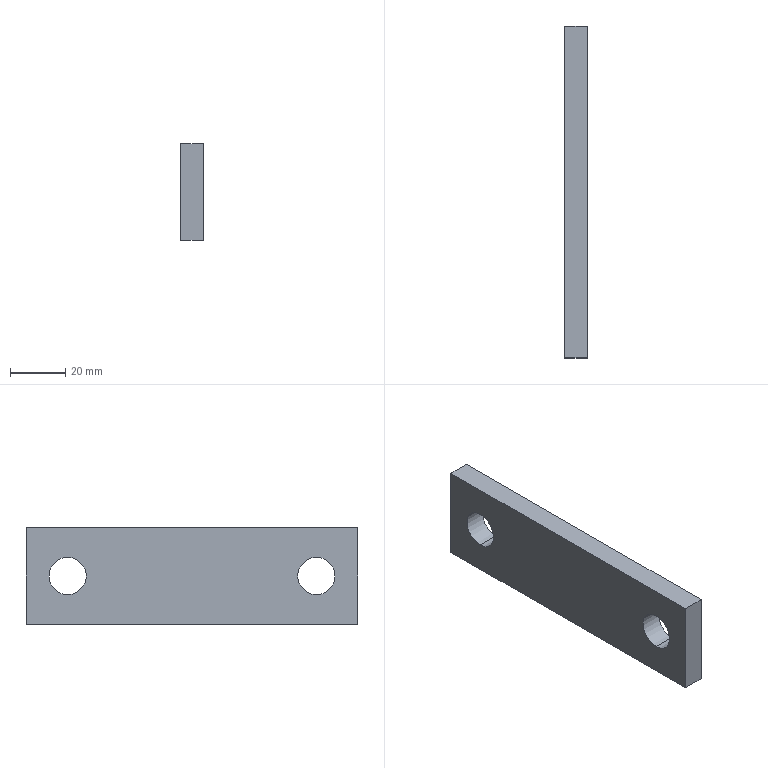Component | SolidWorks | BearingHousing-1_ShaftBaffle-1 | 1 solid | 10 faces | box 8 x 120 x 35 mm | volume 31310 mm3 | plane 6 | cylinder 4 | commonest cylinder face diameters 13.5 x4 | material Plain Carbon Steel
STEP:
#1=CARTESIAN_POINT('',(427.659,129.202,273.063));
#2=VERTEX_POINT('',#1);
#3=CARTESIAN_POINT('',(427.659,129.202,273.594));
#4=VERTEX_POINT('',#3);
#5=CARTESIAN_POINT('',(427.659,129.202,273.328));
#6=DIRECTION('',(-1.,-0.,0.));
#7=DIRECTION('',(0.,0.,1.));
#8=AXIS2_PLACEMENT_3D('',#5,#6,#7);
#9=CIRCLE('',#8,0.2657);
#10=EDGE_CURVE('',#2,#4,#9,.T.);
#11=ORIENTED_EDGE('',*,*,#10,.F.);
#12=CARTESIAN_POINT('',(427.344,129.202,273.063));
#13=VERTEX_POINT('',#12);
#14=CARTESIAN_POINT('',(427.659,129.202,273.063));
#15=DIRECTION('',(-1.,-0.,0.));
#16=VECTOR('',#15,39.37);
#17=LINE('',#14,#16);
#18=EDGE_CURVE('',#2,#13,#17,.T.);
#19=ORIENTED_EDGE('',*,*,#18,.T.);
#20=CARTESIAN_POINT('',(427.344,129.202,273.594));
#21=VERTEX_POINT('',#20);
#22=CARTESIAN_POINT('',(427.344,129.202,273.328));
#23=DIRECTION('',(-1.,-0.,0.));
#24=DIRECTION('',(0.,0.,1.));
#25=AXIS2_PLACEMENT_3D('',#22,#23,#24);
#26=CIRCLE('',#25,0.2657);
#27=EDGE_CURVE('',#13,#21,#26,.T.);
#28=ORIENTED_EDGE('',*,*,#27,.T.);
#29=CARTESIAN_POINT('',(427.659,129.202,273.594));
#30=DIRECTION('',(-1.,-0.,0.));
#31=VECTOR('',#30,39.37);
#32=LINE('',#29,#31);
#33=EDGE_CURVE('',#4,#21,#32,.T.);
#34=ORIENTED_EDGE('',*,*,#33,.F.);
#35=EDGE_LOOP('',(#11,#19,#28,#34));
#36=FACE_OUTER_BOUND('',#35,.T.);
#37=CARTESIAN_POINT('',(427.659,129.202,273.328));
#38=DIRECTION('',(-1.,-0.,0.));
#39=DIRECTION('',(0.,0.,1.));
#40=AXIS2_PLACEMENT_3D('',#37,#38,#39);
#41=CYLINDRICAL_SURFACE('',#40,0.2657);
#42=ADVANCED_FACE('',(#36),#41,.F.);
#43=CARTESIAN_POINT('',(427.659,125.659,273.063));
#44=VERTEX_POINT('',#43);
#45=CARTESIAN_POINT('',(427.659,125.659,273.594));
#46=VERTEX_POINT('',#45);
#47=CARTESIAN_POINT('',(427.659,125.659,273.328));
#48=DIRECTION('',(-1.,-0.,0.));
#49=DIRECTION('',(0.,0.,1.));
#50=AXIS2_PLACEMENT_3D('',#47,#48,#49);
#51=CIRCLE('',#50,0.2657);
#52=EDGE_CURVE('',#44,#46,#51,.T.);
#53=ORIENTED_EDGE('',*,*,#52,.F.);
#54=CARTESIAN_POINT('',(427.344,125.659,273.063));
#55=VERTEX_POINT('',#54);
#56=CARTESIAN_POINT('',(427.659,125.659,273.063));
#57=DIRECTION('',(-1.,-0.,0.));
#58=VECTOR('',#57,39.37);
#59=LINE('',#56,#58);
#60=EDGE_CURVE('',#44,#55,#59,.T.);
#61=ORIENTED_EDGE('',*,*,#60,.T.);
#62=CARTESIAN_POINT('',(427.344,125.659,273.594));
#63=VERTEX_POINT('',#62);
#64=CARTESIAN_POINT('',(427.344,125.659,273.328));
#65=DIRECTION('',(-1.,-0.,0.));
#66=DIRECTION('',(0.,0.,1.));
#67=AXIS2_PLACEMENT_3D('',#64,#65,#66);
#68=CIRCLE('',#67,0.2657);
#69=EDGE_CURVE('',#55,#63,#68,.T.);
#70=ORIENTED_EDGE('',*,*,#69,.T.);
#71=CARTESIAN_POINT('',(427.659,125.659,273.594));
#72=DIRECTION('',(-1.,-0.,0.));
#73=VECTOR('',#72,39.37);
#74=LINE('',#71,#73);
#75=EDGE_CURVE('',#46,#63,#74,.T.);
#76=ORIENTED_EDGE('',*,*,#75,.F.);
#77=EDGE_LOOP('',(#53,#61,#70,#76));
#78=FACE_OUTER_BOUND('',#77,.T.);
#79=CARTESIAN_POINT('',(427.659,125.659,273.328));
#80=DIRECTION('',(-1.,-0.,0.));
#81=DIRECTION('',(0.,0.,1.));
#82=AXIS2_PLACEMENT_3D('',#79,#80,#81);
#83=CYLINDRICAL_SURFACE('',#82,0.2657);
#84=ADVANCED_FACE('',(#78),#83,.F.);
#85=CARTESIAN_POINT('',(427.344,125.068,272.639));
#86=VERTEX_POINT('',#85);
#87=CARTESIAN_POINT('',(427.344,125.068,274.017));
#88=VERTEX_POINT('',#87);
#89=CARTESIAN_POINT('',(427.344,125.068,272.639));
#90=DIRECTION('',(-0.,0.,1.));
#91=VECTOR('',#90,39.37);
#92=LINE('',#89,#91);
#93=EDGE_CURVE('',#86,#88,#92,.T.);
#94=ORIENTED_EDGE('',*,*,#93,.F.);
#95=CARTESIAN_POINT('',(427.659,125.068,272.639));
#96=VERTEX_POINT('',#95);
#97=CARTESIAN_POINT('',(427.659,125.068,272.639));
#98=DIRECTION('',(-1.,-0.,0.));
#99=VECTOR('',#98,39.37);
#100=LINE('',#97,#99);
#101=EDGE_CURVE('',#96,#86,#100,.T.);
#102=ORIENTED_EDGE('',*,*,#101,.F.);
#103=CARTESIAN_POINT('',(427.659,125.068,274.017));
#104=VERTEX_POINT('',#103);
#105=CARTESIAN_POINT('',(427.659,125.068,272.639));
#106=DIRECTION('',(-0.,0.,1.));
#107=VECTOR('',#106,39.37);
#108=LINE('',#105,#107);
#109=EDGE_CURVE('',#96,#104,#108,.T.);
#110=ORIENTED_EDGE('',*,*,#109,.T.);
#111=CARTESIAN_POINT('',(427.659,125.068,274.017));
#112=DIRECTION('',(-1.,-0.,0.));
#113=VECTOR('',#112,39.37);
#114=LINE('',#111,#113);
#115=EDGE_CURVE('',#104,#88,#114,.T.);
#116=ORIENTED_EDGE('',*,*,#115,.T.);
#117=EDGE_LOOP('',(#94,#102,#110,#116));
#118=FACE_OUTER_BOUND('',#117,.T.);
#119=CARTESIAN_POINT('',(427.659,125.068,272.639));
#120=DIRECTION('',(0.,-1.,0.));
#121=DIRECTION('',(-0.,0.,1.));
#122=AXIS2_PLACEMENT_3D('',#119,#120,#121);
#123=PLANE('',#122);
#124=ADVANCED_FACE('',(#118),#123,.T.);
#125=CARTESIAN_POINT('',(427.344,129.793,272.639));
#126=VERTEX_POINT('',#125);
#127=CARTESIAN_POINT('',(427.344,125.068,272.639));
#128=DIRECTION('',(0.,-1.,0.));
#129=VECTOR('',#128,39.37);
#130=LINE('',#127,#129);
#131=EDGE_CURVE('',#126,#86,#130,.T.);
#132=ORIENTED_EDGE('',*,*,#131,.F.);
#133=CARTESIAN_POINT('',(427.659,129.793,272.639));
#134=VERTEX_POINT('',#133);
#135=CARTESIAN_POINT('',(427.659,129.793,272.639));
#136=DIRECTION('',(-1.,-0.,0.));
#137=VECTOR('',#136,39.37);
#138=LINE('',#135,#137);
#139=EDGE_CURVE('',#134,#126,#138,.T.);
#140=ORIENTED_EDGE('',*,*,#139,.F.);
#141=CARTESIAN_POINT('',(427.659,125.068,272.639));
#142=DIRECTION('',(0.,-1.,0.));
#143=VECTOR('',#142,39.37);
#144=LINE('',#141,#143);
#145=EDGE_CURVE('',#134,#96,#144,.T.);
#146=ORIENTED_EDGE('',*,*,#145,.T.);
#147=ORIENTED_EDGE('',*,*,#101,.T.);
#148=EDGE_LOOP('',(#132,#140,#146,#147));
#149=FACE_OUTER_BOUND('',#148,.T.);
#150=CARTESIAN_POINT('',(427.659,125.068,272.639));
#151=DIRECTION('',(0.,0.,-1.));
#152=DIRECTION('',(0.,-1.,0.));
#153=AXIS2_PLACEMENT_3D('',#150,#151,#152);
#154=PLANE('',#153);
#155=ADVANCED_FACE('',(#149),#154,.T.);
#156=CARTESIAN_POINT('',(427.344,129.793,274.017));
#157=VERTEX_POINT('',#156);
#158=CARTESIAN_POINT('',(427.344,129.793,272.639));
#159=DIRECTION('',(0.,0.,-1.));
#160=VECTOR('',#159,39.37);
#161=LINE('',#158,#160);
#162=EDGE_CURVE('',#157,#126,#161,.T.);
#163=ORIENTED_EDGE('',*,*,#162,.F.);
#164=CARTESIAN_POINT('',(427.659,129.793,274.017));
#165=VERTEX_POINT('',#164);
#166=CARTESIAN_POINT('',(427.659,129.793,274.017));
#167=DIRECTION('',(-1.,-0.,0.));
#168=VECTOR('',#167,39.37);
#169=LINE('',#166,#168);
#170=EDGE_CURVE('',#165,#157,#169,.T.);
#171=ORIENTED_EDGE('',*,*,#170,.F.);
#172=CARTESIAN_POINT('',(427.659,129.793,272.639));
#173=DIRECTION('',(0.,0.,-1.));
#174=VECTOR('',#173,39.37);
#175=LINE('',#172,#174);
#176=EDGE_CURVE('',#165,#134,#175,.T.);
#177=ORIENTED_EDGE('',*,*,#176,.T.);
#178=ORIENTED_EDGE('',*,*,#139,.T.);
#179=EDGE_LOOP('',(#163,#171,#177,#178));
#180=FACE_OUTER_BOUND('',#179,.T.);
#181=CARTESIAN_POINT('',(427.659,129.793,272.639));
#182=DIRECTION('',(-0.,1.,0.));
#183=DIRECTION('',(0.,0.,-1.));
#184=AXIS2_PLACEMENT_3D('',#181,#182,#183);
#185=PLANE('',#184);
#186=ADVANCED_FACE('',(#180),#185,.T.);
#187=CARTESIAN_POINT('',(427.344,125.068,274.017));
#188=DIRECTION('',(-0.,1.,0.));
#189=VECTOR('',#188,39.37);
#190=LINE('',#187,#189);
#191=EDGE_CURVE('',#88,#157,#190,.T.);
#192=ORIENTED_EDGE('',*,*,#191,.F.);
#193=ORIENTED_EDGE('',*,*,#115,.F.);
#194=CARTESIAN_POINT('',(427.659,125.068,274.017));
#195=DIRECTION('',(-0.,1.,0.));
#196=VECTOR('',#195,39.37);
#197=LINE('',#194,#196);
#198=EDGE_CURVE('',#104,#165,#197,.T.);
#199=ORIENTED_EDGE('',*,*,#198,.T.);
#200=ORIENTED_EDGE('',*,*,#170,.T.);
#201=EDGE_LOOP('',(#192,#193,#199,#200));
#202=FACE_OUTER_BOUND('',#201,.T.);
#203=CARTESIAN_POINT('',(427.659,125.068,274.017));
#204=DIRECTION('',(0.,0.,1.));
#205=DIRECTION('',(-0.,1.,0.));
#206=AXIS2_PLACEMENT_3D('',#203,#204,#205);
#207=PLANE('',#206);
#208=ADVANCED_FACE('',(#202),#207,.T.);
#209=CARTESIAN_POINT('',(427.659,129.202,273.328));
#210=DIRECTION('',(-1.,-0.,0.));
#211=DIRECTION('',(0.,0.,1.));
#212=AXIS2_PLACEMENT_3D('',#209,#210,#211);
#213=CIRCLE('',#212,0.2657);
#214=EDGE_CURVE('',#4,#2,#213,.T.);
#215=ORIENTED_EDGE('',*,*,#214,.T.);
#216=ORIENTED_EDGE('',*,*,#10,.T.);
#217=EDGE_LOOP('',(#215,#216));
#218=FACE_BOUND('',#217,.T.);
#219=CARTESIAN_POINT('',(427.659,125.659,273.328));
#220=DIRECTION('',(-1.,-0.,0.));
#221=DIRECTION('',(0.,0.,1.));
#222=AXIS2_PLACEMENT_3D('',#219,#220,#221);
#223=CIRCLE('',#222,0.2657);
#224=EDGE_CURVE('',#46,#44,#223,.T.);
#225=ORIENTED_EDGE('',*,*,#224,.T.);
#226=ORIENTED_EDGE('',*,*,#52,.T.);
#227=EDGE_LOOP('',(#225,#226));
#228=FACE_BOUND('',#227,.T.);
#229=ORIENTED_EDGE('',*,*,#109,.F.);
#230=ORIENTED_EDGE('',*,*,#145,.F.);
#231=ORIENTED_EDGE('',*,*,#176,.F.);
#232=ORIENTED_EDGE('',*,*,#198,.F.);
#233=EDGE_LOOP('',(#229,#230,#231,#232));
#234=FACE_OUTER_BOUND('',#233,.T.);
#235=CARTESIAN_POINT('',(427.659,125.068,272.639));
#236=DIRECTION('',(-1.,-0.,0.));
#237=DIRECTION('',(0.,0.,1.));
#238=AXIS2_PLACEMENT_3D('',#235,#236,#237);
#239=PLANE('',#238);
#240=ADVANCED_FACE('',(#218,#228,#234),#239,.F.);
#241=CARTESIAN_POINT('',(427.344,129.202,273.328));
#242=DIRECTION('',(-1.,-0.,0.));
#243=DIRECTION('',(0.,0.,1.));
#244=AXIS2_PLACEMENT_3D('',#241,#242,#243);
#245=CIRCLE('',#244,0.2657);
#246=EDGE_CURVE('',#21,#13,#245,.T.);
#247=ORIENTED_EDGE('',*,*,#246,.F.);
#248=ORIENTED_EDGE('',*,*,#27,.F.);
#249=EDGE_LOOP('',(#247,#248));
#250=FACE_BOUND('',#249,.T.);
#251=CARTESIAN_POINT('',(427.344,125.659,273.328));
#252=DIRECTION('',(-1.,-0.,0.));
#253=DIRECTION('',(0.,0.,1.));
#254=AXIS2_PLACEMENT_3D('',#251,#252,#253);
#255=CIRCLE('',#254,0.2657);
#256=EDGE_CURVE('',#63,#55,#255,.T.);
#257=ORIENTED_EDGE('',*,*,#256,.F.);
#258=ORIENTED_EDGE('',*,*,#69,.F.);
#259=EDGE_LOOP('',(#257,#258));
#260=FACE_BOUND('',#259,.T.);
#261=ORIENTED_EDGE('',*,*,#93,.T.);
#262=ORIENTED_EDGE('',*,*,#191,.T.);
#263=ORIENTED_EDGE('',*,*,#162,.T.);
#264=ORIENTED_EDGE('',*,*,#131,.T.);
#265=EDGE_LOOP('',(#261,#262,#263,#264));
#266=FACE_OUTER_BOUND('',#265,.T.);
#267=CARTESIAN_POINT('',(427.344,125.068,272.639));
#268=DIRECTION('',(-1.,-0.,0.));
#269=DIRECTION('',(0.,0.,1.));
#270=AXIS2_PLACEMENT_3D('',#267,#268,#269);
#271=PLANE('',#270);
#272=ADVANCED_FACE('',(#250,#260,#266),#271,.T.);
#273=ORIENTED_EDGE('',*,*,#60,.F.);
#274=ORIENTED_EDGE('',*,*,#224,.F.);
#275=ORIENTED_EDGE('',*,*,#75,.T.);
#276=ORIENTED_EDGE('',*,*,#256,.T.);
#277=EDGE_LOOP('',(#273,#274,#275,#276));
#278=FACE_OUTER_BOUND('',#277,.T.);
#279=CARTESIAN_POINT('',(427.659,125.659,273.328));
#280=DIRECTION('',(-1.,-0.,0.));
#281=DIRECTION('',(0.,0.,1.));
#282=AXIS2_PLACEMENT_3D('',#279,#280,#281);
#283=CYLINDRICAL_SURFACE('',#282,0.2657);
#284=ADVANCED_FACE('',(#278),#283,.F.);
#285=ORIENTED_EDGE('',*,*,#18,.F.);
#286=ORIENTED_EDGE('',*,*,#214,.F.);
#287=ORIENTED_EDGE('',*,*,#33,.T.);
#288=ORIENTED_EDGE('',*,*,#246,.T.);
#289=EDGE_LOOP('',(#285,#286,#287,#288));
#290=FACE_OUTER_BOUND('',#289,.T.);
#291=CARTESIAN_POINT('',(427.659,129.202,273.328));
#292=DIRECTION('',(-1.,-0.,0.));
#293=DIRECTION('',(0.,0.,1.));
#294=AXIS2_PLACEMENT_3D('',#291,#292,#293);
#295=CYLINDRICAL_SURFACE('',#294,0.2657);
#296=ADVANCED_FACE('',(#290),#295,.F.);
#297=CLOSED_SHELL('',(#42,#84,#124,#155,#186,#208,#240,#272,#284,#296));
#298=MANIFOLD_SOLID_BREP('',#297);
#299=CARTESIAN_POINT('',(0.,0.,0.));
#300=DIRECTION('',(0.,0.,1.));
#301=DIRECTION('',(1.,0.,0.));
#302=AXIS2_PLACEMENT_3D('',#299,#300,#301);
#303=(LENGTH_UNIT()NAMED_UNIT(*)SI_UNIT($,.METRE.));
#304=LENGTH_MEASURE_WITH_UNIT(LENGTH_MEASURE(0.0254),#303);
#305=DIMENSIONAL_EXPONENTS(1.,0.,0.,0.,0.,0.,0.);
#306=(CONVERSION_BASED_UNIT('',#304)LENGTH_UNIT()NAMED_UNIT(#305));
#307=UNCERTAINTY_MEASURE_WITH_UNIT(LENGTH_MEASURE(0.00001),#306,'','');
#308=(NAMED_UNIT(*)PLANE_ANGLE_UNIT()SI_UNIT($,.RADIAN.));
#309=(NAMED_UNIT(*)SI_UNIT($,.STERADIAN.)SOLID_ANGLE_UNIT());
#310=(GEOMETRIC_REPRESENTATION_CONTEXT(3)GLOBAL_UNCERTAINTY_ASSIGNED_CONTEXT((#307))GLOBAL_UNIT_ASSIGNED_CONTEXT((#306,#308,#309))REPRESENTATION_CONTEXT('',''));
#311=ADVANCED_BREP_SHAPE_REPRESENTATION('',(#298,#302),#310);
#312=COLOUR_RGB('',0.7922,0.8196,0.9333);
#313=FILL_AREA_STYLE_COLOUR('',#312);
#314=FILL_AREA_STYLE('',(#313));
#315=SURFACE_STYLE_FILL_AREA(#314);
#316=SURFACE_SIDE_STYLE('',(#315));
#317=SURFACE_STYLE_USAGE(.BOTH.,#316);
#318=PRESENTATION_STYLE_ASSIGNMENT((#317));
#319=STYLED_ITEM('',(#318),#298);
#320=PRESENTATION_LAYER_ASSIGNMENT('','',(#319));
#321=(LENGTH_UNIT()NAMED_UNIT(*)SI_UNIT($,.METRE.));
#322=LENGTH_MEASURE_WITH_UNIT(LENGTH_MEASURE(0.0254),#321);
#323=DIMENSIONAL_EXPONENTS(1.,0.,0.,0.,0.,0.,0.);
#324=(CONVERSION_BASED_UNIT('',#322)LENGTH_UNIT()NAMED_UNIT(#323));
#325=UNCERTAINTY_MEASURE_WITH_UNIT(LENGTH_MEASURE(0.00001),#324,'','');
#326=(NAMED_UNIT(*)PLANE_ANGLE_UNIT()SI_UNIT($,.RADIAN.));
#327=(NAMED_UNIT(*)SI_UNIT($,.STERADIAN.)SOLID_ANGLE_UNIT());
#328=(GEOMETRIC_REPRESENTATION_CONTEXT(3)GLOBAL_UNCERTAINTY_ASSIGNED_CONTEXT((#325))GLOBAL_UNIT_ASSIGNED_CONTEXT((#324,#326,#327))REPRESENTATION_CONTEXT('',''));
#329=MECHANICAL_DESIGN_GEOMETRIC_PRESENTATION_REPRESENTATION('',(#319),#328);